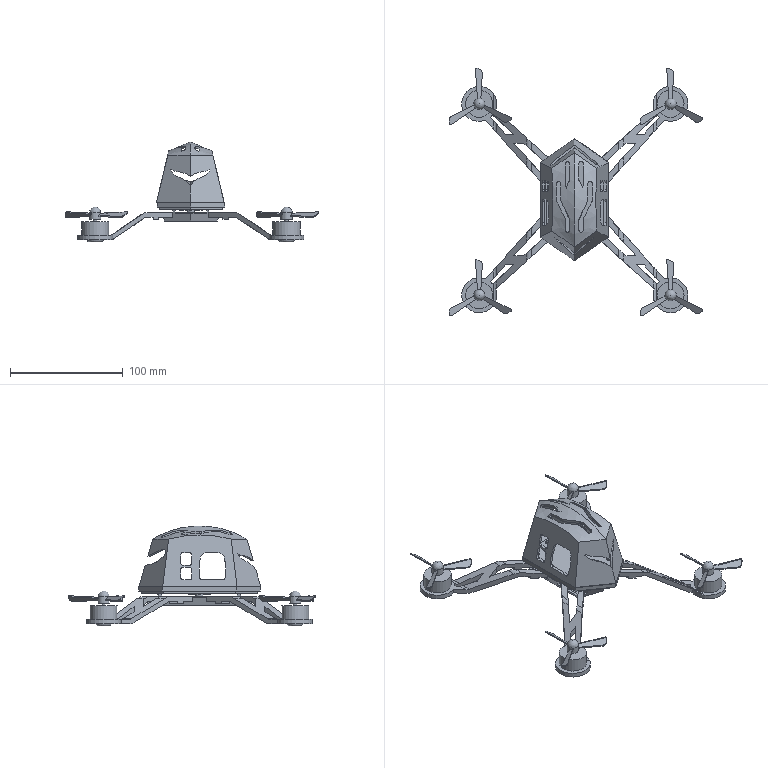Assembly | NX | mm | 17 component files | 37 solids | 586 faces | box 225.26 x 219.83 x 88.78 mm | volume 120824 mm3 | plane 366 | cylinder 194 | spline 18 | torus 4 | sphere 4 | commonest cylinder face diameters 4 x34 10 x26 8 x22 16 x18 3 x17 2 x12 31 x8 14 x8
Bill of materials:
unnamed part 1 | 4 |  | Stepped, rotationally symmetric part: a short large-diameter cylindrical disk with a smaller coaxial cylindrical boss on one side; the boss has a rounded end edge. A small hole sits at the center of the large flat face.
unnamed part 2 | 1 |  | Thin flat rectangular plate with four chamfered corners and six through holes: two larger holes on the centerline near the short edges and four smaller holes near the corners.
unnamed part 3 | 4 |  | Three-blade propeller-like rotor: a cylindrical hub with a domed cap, three flat tapered blades radiating at roughly equal spacing and tilted relative to the hub plane, and a slender cylindrical shaft extending from the underside of the hub.
unnamed part 4 | 1 |  | Hollow faceted shell with an elongated pointed-hexagon footprint, tapered side walls and a curved crowned top. Decorative/vent cutouts go through the walls: a wing-shaped cutout on one end face, a large rounded-rectangle window and two smaller square windows on a side face, curved slots on the angled faces, and Y-shaped and straight slots on the top.
unnamed part 5 | 1 |  | Shallow tray/base with an elongated hexagonal outline: a thin floor, a low sloped perimeter lip, several upright rectangular tabs/walls along the edges, and a central cylindrical boss with a hole, braced by four thin radial ribs in a cross pattern.
unnamed part 6 | 1 |  | Flat plate with an elongated hexagonal outline (pointed ends), six holes (two larger on the long centerline, four smaller in a rectangular pattern), a stepped underside edge, and a small cylindrical boss/pin protruding from the center of the underside.
unnamed part 7 | 4 |  | Symmetric stepped cylindrical pin: a central larger-diameter collar with equal smaller-diameter cylindrical sections extending from both sides, sharing one axis.
unnamed part 8 | 1 |  | X-shaped open frame: four truss-style arms with cross bracing run from a central ring with a large circular opening to four annular pads, each with a central hole. The arms bend so the center sits higher than the end pads. Two small eared tabs with small holes project from the central ring.
Mates:
1. align lock | base_plate 1 edge | shell 1 edge
2. concentric | bracket 1 edge | base_plate 1 edge
3. concentric | cover_plate 1 edge | base_plate 1 edge
4. concentric | motor_mount 4 edge | bracket 1 edge
5. concentric | propeller 4 edge | motor_mount 4 edge
6. concentric | motor_mount 3 edge | bracket 1 edge
7. concentric | motor_mount 2 edge | bracket 1 edge
8. concentric | motor_mount 1 edge | bracket 1 edge
9. concentric | propeller 3 edge | motor_mount 3 edge
10. concentric | propeller 2 edge | motor_mount 2 edge
11. concentric | propeller 1 edge | motor_mount 1 edge
12. concentric | plate 1 edge | base_plate 1 edge
13. concentric | circuit_pin 4 edge | plate 1 edge